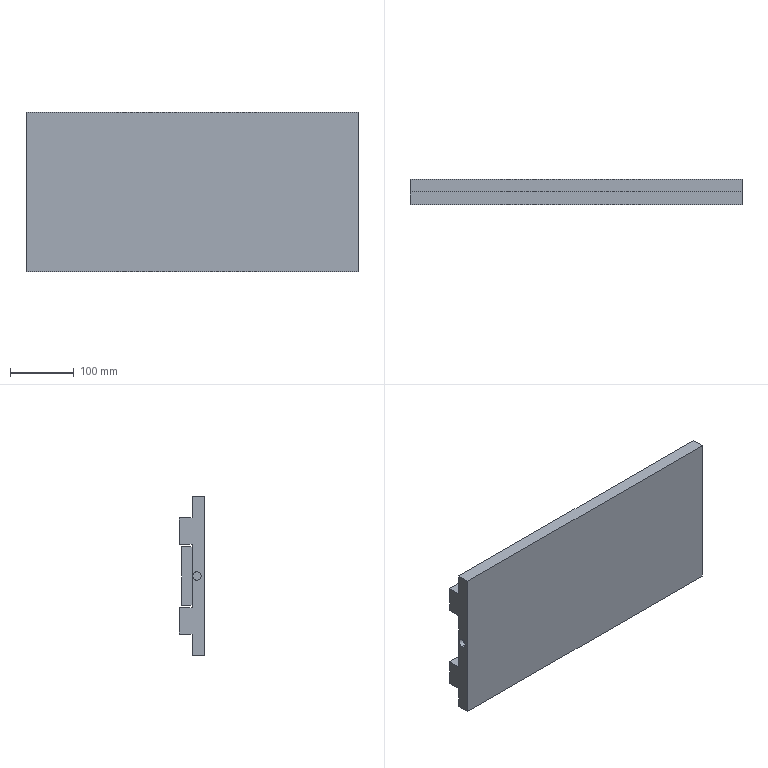Component | SolidWorks | X-AxisSupportBase-1 | 1 solid | 38 faces | box 520 x 40 x 250 mm | volume 3501982 mm3 | plane 26 | cylinder 12 | commonest cylinder face diameters 5.084 x8 13.093 x2 2.946 x2
STEP:
#1=COLOUR_RGB('',0.7922,0.8196,0.9333);
#2=FILL_AREA_STYLE_COLOUR('',#1);
#3=FILL_AREA_STYLE('',(#2));
#4=SURFACE_STYLE_FILL_AREA(#3);
#5=SURFACE_SIDE_STYLE('',(#4));
#6=SURFACE_STYLE_USAGE(.BOTH.,#5);
#7=PRESENTATION_STYLE_ASSIGNMENT((#6));
#8=CARTESIAN_POINT('',(6.767,1.417,1.368));
#9=VERTEX_POINT('',#8);
#10=CARTESIAN_POINT('',(6.767,1.417,1.568));
#11=VERTEX_POINT('',#10);
#12=CARTESIAN_POINT('',(6.767,1.417,1.468));
#13=DIRECTION('',(0.,1.,0.));
#14=DIRECTION('',(0.,0.,1.));
#15=AXIS2_PLACEMENT_3D('',#12,#13,#14);
#16=CIRCLE('',#15,0.1001);
#17=EDGE_CURVE('',#9,#11,#16,.T.);
#18=ORIENTED_EDGE('',*,*,#17,.T.);
#19=CARTESIAN_POINT('',(6.767,0.7874,1.568));
#20=VERTEX_POINT('',#19);
#21=CARTESIAN_POINT('',(6.767,1.417,1.568));
#22=DIRECTION('',(0.,-1.,0.));
#23=VECTOR('',#22,39.37);
#24=LINE('',#21,#23);
#25=EDGE_CURVE('',#11,#20,#24,.T.);
#26=ORIENTED_EDGE('',*,*,#25,.T.);
#27=CARTESIAN_POINT('',(6.767,0.7874,1.368));
#28=VERTEX_POINT('',#27);
#29=CARTESIAN_POINT('',(6.767,0.7874,1.468));
#30=DIRECTION('',(0.,1.,0.));
#31=DIRECTION('',(0.,0.,1.));
#32=AXIS2_PLACEMENT_3D('',#29,#30,#31);
#33=CIRCLE('',#32,0.1001);
#34=EDGE_CURVE('',#28,#20,#33,.T.);
#35=ORIENTED_EDGE('',*,*,#34,.F.);
#36=CARTESIAN_POINT('',(6.767,1.417,1.368));
#37=DIRECTION('',(0.,-1.,0.));
#38=VECTOR('',#37,39.37);
#39=LINE('',#36,#38);
#40=EDGE_CURVE('',#9,#28,#39,.T.);
#41=ORIENTED_EDGE('',*,*,#40,.F.);
#42=EDGE_LOOP('',(#18,#26,#35,#41));
#43=FACE_OUTER_BOUND('',#42,.T.);
#44=CARTESIAN_POINT('',(6.767,1.417,1.468));
#45=DIRECTION('',(0.,-1.,0.));
#46=DIRECTION('',(0.,0.,-1.));
#47=AXIS2_PLACEMENT_3D('',#44,#45,#46);
#48=CYLINDRICAL_SURFACE('',#47,0.1001);
#49=ADVANCED_FACE('',(#43),#48,.F.);
#50=CARTESIAN_POINT('',(6.208,1.417,1.368));
#51=VERTEX_POINT('',#50);
#52=CARTESIAN_POINT('',(6.208,1.417,1.568));
#53=VERTEX_POINT('',#52);
#54=CARTESIAN_POINT('',(6.208,1.417,1.468));
#55=DIRECTION('',(0.,1.,0.));
#56=DIRECTION('',(0.,0.,1.));
#57=AXIS2_PLACEMENT_3D('',#54,#55,#56);
#58=CIRCLE('',#57,0.1001);
#59=EDGE_CURVE('',#51,#53,#58,.T.);
#60=ORIENTED_EDGE('',*,*,#59,.T.);
#61=CARTESIAN_POINT('',(6.208,0.7874,1.568));
#62=VERTEX_POINT('',#61);
#63=CARTESIAN_POINT('',(6.208,1.417,1.568));
#64=DIRECTION('',(0.,-1.,0.));
#65=VECTOR('',#64,39.37);
#66=LINE('',#63,#65);
#67=EDGE_CURVE('',#53,#62,#66,.T.);
#68=ORIENTED_EDGE('',*,*,#67,.T.);
#69=CARTESIAN_POINT('',(6.208,0.7874,1.368));
#70=VERTEX_POINT('',#69);
#71=CARTESIAN_POINT('',(6.208,0.7874,1.468));
#72=DIRECTION('',(0.,1.,0.));
#73=DIRECTION('',(0.,0.,1.));
#74=AXIS2_PLACEMENT_3D('',#71,#72,#73);
#75=CIRCLE('',#74,0.1001);
#76=EDGE_CURVE('',#70,#62,#75,.T.);
#77=ORIENTED_EDGE('',*,*,#76,.F.);
#78=CARTESIAN_POINT('',(6.208,1.417,1.368));
#79=DIRECTION('',(0.,-1.,0.));
#80=VECTOR('',#79,39.37);
#81=LINE('',#78,#80);
#82=EDGE_CURVE('',#51,#70,#81,.T.);
#83=ORIENTED_EDGE('',*,*,#82,.F.);
#84=EDGE_LOOP('',(#60,#68,#77,#83));
#85=FACE_OUTER_BOUND('',#84,.T.);
#86=CARTESIAN_POINT('',(6.208,1.417,1.468));
#87=DIRECTION('',(0.,-1.,0.));
#88=DIRECTION('',(0.,0.,-1.));
#89=AXIS2_PLACEMENT_3D('',#86,#87,#88);
#90=CYLINDRICAL_SURFACE('',#89,0.1001);
#91=ADVANCED_FACE('',(#85),#90,.F.);
#92=CARTESIAN_POINT('',(6.767,1.417,-1.568));
#93=VERTEX_POINT('',#92);
#94=CARTESIAN_POINT('',(6.767,1.417,-1.368));
#95=VERTEX_POINT('',#94);
#96=CARTESIAN_POINT('',(6.767,1.417,-1.468));
#97=DIRECTION('',(0.,1.,0.));
#98=DIRECTION('',(0.,0.,1.));
#99=AXIS2_PLACEMENT_3D('',#96,#97,#98);
#100=CIRCLE('',#99,0.1001);
#101=EDGE_CURVE('',#93,#95,#100,.T.);
#102=ORIENTED_EDGE('',*,*,#101,.T.);
#103=CARTESIAN_POINT('',(6.767,0.7874,-1.368));
#104=VERTEX_POINT('',#103);
#105=CARTESIAN_POINT('',(6.767,1.417,-1.368));
#106=DIRECTION('',(0.,-1.,0.));
#107=VECTOR('',#106,39.37);
#108=LINE('',#105,#107);
#109=EDGE_CURVE('',#95,#104,#108,.T.);
#110=ORIENTED_EDGE('',*,*,#109,.T.);
#111=CARTESIAN_POINT('',(6.767,0.7874,-1.568));
#112=VERTEX_POINT('',#111);
#113=CARTESIAN_POINT('',(6.767,0.7874,-1.468));
#114=DIRECTION('',(0.,1.,0.));
#115=DIRECTION('',(0.,0.,1.));
#116=AXIS2_PLACEMENT_3D('',#113,#114,#115);
#117=CIRCLE('',#116,0.1001);
#118=EDGE_CURVE('',#112,#104,#117,.T.);
#119=ORIENTED_EDGE('',*,*,#118,.F.);
#120=CARTESIAN_POINT('',(6.767,1.417,-1.568));
#121=DIRECTION('',(0.,-1.,0.));
#122=VECTOR('',#121,39.37);
#123=LINE('',#120,#122);
#124=EDGE_CURVE('',#93,#112,#123,.T.);
#125=ORIENTED_EDGE('',*,*,#124,.F.);
#126=EDGE_LOOP('',(#102,#110,#119,#125));
#127=FACE_OUTER_BOUND('',#126,.T.);
#128=CARTESIAN_POINT('',(6.767,1.417,-1.468));
#129=DIRECTION('',(0.,-1.,0.));
#130=DIRECTION('',(0.,0.,-1.));
#131=AXIS2_PLACEMENT_3D('',#128,#129,#130);
#132=CYLINDRICAL_SURFACE('',#131,0.1001);
#133=ADVANCED_FACE('',(#127),#132,.F.);
#134=CARTESIAN_POINT('',(6.208,1.417,-1.568));
#135=VERTEX_POINT('',#134);
#136=CARTESIAN_POINT('',(6.208,1.417,-1.368));
#137=VERTEX_POINT('',#136);
#138=CARTESIAN_POINT('',(6.208,1.417,-1.468));
#139=DIRECTION('',(0.,1.,0.));
#140=DIRECTION('',(0.,0.,1.));
#141=AXIS2_PLACEMENT_3D('',#138,#139,#140);
#142=CIRCLE('',#141,0.1001);
#143=EDGE_CURVE('',#135,#137,#142,.T.);
#144=ORIENTED_EDGE('',*,*,#143,.T.);
#145=CARTESIAN_POINT('',(6.208,0.7874,-1.368));
#146=VERTEX_POINT('',#145);
#147=CARTESIAN_POINT('',(6.208,1.417,-1.368));
#148=DIRECTION('',(0.,-1.,0.));
#149=VECTOR('',#148,39.37);
#150=LINE('',#147,#149);
#151=EDGE_CURVE('',#137,#146,#150,.T.);
#152=ORIENTED_EDGE('',*,*,#151,.T.);
#153=CARTESIAN_POINT('',(6.208,0.7874,-1.568));
#154=VERTEX_POINT('',#153);
#155=CARTESIAN_POINT('',(6.208,0.7874,-1.468));
#156=DIRECTION('',(0.,1.,0.));
#157=DIRECTION('',(0.,0.,1.));
#158=AXIS2_PLACEMENT_3D('',#155,#156,#157);
#159=CIRCLE('',#158,0.1001);
#160=EDGE_CURVE('',#154,#146,#159,.T.);
#161=ORIENTED_EDGE('',*,*,#160,.F.);
#162=CARTESIAN_POINT('',(6.208,1.417,-1.568));
#163=DIRECTION('',(0.,-1.,0.));
#164=VECTOR('',#163,39.37);
#165=LINE('',#162,#164);
#166=EDGE_CURVE('',#135,#154,#165,.T.);
#167=ORIENTED_EDGE('',*,*,#166,.F.);
#168=EDGE_LOOP('',(#144,#152,#161,#167));
#169=FACE_OUTER_BOUND('',#168,.T.);
#170=CARTESIAN_POINT('',(6.208,1.417,-1.468));
#171=DIRECTION('',(0.,-1.,0.));
#172=DIRECTION('',(0.,0.,-1.));
#173=AXIS2_PLACEMENT_3D('',#170,#171,#172);
#174=CYLINDRICAL_SURFACE('',#173,0.1001);
#175=ADVANCED_FACE('',(#169),#174,.F.);
#176=CARTESIAN_POINT('',(-10.591,0.4812,-0.2577));
#177=VERTEX_POINT('',#176);
#178=CARTESIAN_POINT('',(-10.591,0.4812,0.2577));
#179=VERTEX_POINT('',#178);
#180=CARTESIAN_POINT('',(-10.591,0.4812,0.));
#181=DIRECTION('',(-1.,0.,0.));
#182=DIRECTION('',(0.,0.,1.));
#183=AXIS2_PLACEMENT_3D('',#180,#181,#182);
#184=CIRCLE('',#183,0.2577);
#185=EDGE_CURVE('',#177,#179,#184,.T.);
#186=ORIENTED_EDGE('',*,*,#185,.F.);
#187=CARTESIAN_POINT('',(-10.906,0.4812,-0.2577));
#188=VERTEX_POINT('',#187);
#189=CARTESIAN_POINT('',(-10.591,0.4812,-0.2577));
#190=DIRECTION('',(-1.,0.,0.));
#191=VECTOR('',#190,39.37);
#192=LINE('',#189,#191);
#193=EDGE_CURVE('',#177,#188,#192,.T.);
#194=ORIENTED_EDGE('',*,*,#193,.T.);
#195=CARTESIAN_POINT('',(-10.906,0.4812,0.2577));
#196=VERTEX_POINT('',#195);
#197=CARTESIAN_POINT('',(-10.906,0.4812,0.));
#198=DIRECTION('',(-1.,0.,0.));
#199=DIRECTION('',(0.,0.,1.));
#200=AXIS2_PLACEMENT_3D('',#197,#198,#199);
#201=CIRCLE('',#200,0.2577);
#202=EDGE_CURVE('',#188,#196,#201,.T.);
#203=ORIENTED_EDGE('',*,*,#202,.T.);
#204=CARTESIAN_POINT('',(-10.591,0.4812,0.2577));
#205=DIRECTION('',(-1.,0.,0.));
#206=VECTOR('',#205,39.37);
#207=LINE('',#204,#206);
#208=EDGE_CURVE('',#179,#196,#207,.T.);
#209=ORIENTED_EDGE('',*,*,#208,.F.);
#210=EDGE_LOOP('',(#186,#194,#203,#209));
#211=FACE_OUTER_BOUND('',#210,.T.);
#212=CARTESIAN_POINT('',(-10.591,0.4812,0.));
#213=DIRECTION('',(-1.,0.,0.));
#214=DIRECTION('',(0.,0.,1.));
#215=AXIS2_PLACEMENT_3D('',#212,#213,#214);
#216=CYLINDRICAL_SURFACE('',#215,0.2577);
#217=ADVANCED_FACE('',(#211),#216,.F.);
#218=CARTESIAN_POINT('',(-10.906,1.575,3.579));
#219=VERTEX_POINT('',#218);
#220=CARTESIAN_POINT('',(9.567,1.575,3.579));
#221=VERTEX_POINT('',#220);
#222=CARTESIAN_POINT('',(0.,1.575,3.579));
#223=DIRECTION('',(1.,0.,0.));
#224=VECTOR('',#223,39.37);
#225=LINE('',#222,#224);
#226=EDGE_CURVE('',#219,#221,#225,.T.);
#227=ORIENTED_EDGE('',*,*,#226,.T.);
#228=CARTESIAN_POINT('',(9.567,1.575,1.945));
#229=VERTEX_POINT('',#228);
#230=CARTESIAN_POINT('',(9.567,1.575,0.));
#231=DIRECTION('',(0.,0.,-1.));
#232=VECTOR('',#231,39.37);
#233=LINE('',#230,#232);
#234=EDGE_CURVE('',#221,#229,#233,.T.);
#235=ORIENTED_EDGE('',*,*,#234,.T.);
#236=CARTESIAN_POINT('',(-10.906,1.575,1.945));
#237=VERTEX_POINT('',#236);
#238=CARTESIAN_POINT('',(0.,1.575,1.945));
#239=DIRECTION('',(-1.,0.,0.));
#240=VECTOR('',#239,39.37);
#241=LINE('',#238,#240);
#242=EDGE_CURVE('',#229,#237,#241,.T.);
#243=ORIENTED_EDGE('',*,*,#242,.T.);
#244=CARTESIAN_POINT('',(-10.906,1.575,0.));
#245=DIRECTION('',(0.,0.,1.));
#246=VECTOR('',#245,39.37);
#247=LINE('',#244,#246);
#248=EDGE_CURVE('',#237,#219,#247,.T.);
#249=ORIENTED_EDGE('',*,*,#248,.T.);
#250=EDGE_LOOP('',(#227,#235,#243,#249));
#251=FACE_OUTER_BOUND('',#250,.T.);
#252=CARTESIAN_POINT('',(0.,1.575,0.));
#253=DIRECTION('',(0.,1.,0.));
#254=DIRECTION('',(0.,0.,1.));
#255=AXIS2_PLACEMENT_3D('',#252,#253,#254);
#256=PLANE('',#255);
#257=ADVANCED_FACE('',(#251),#256,.T.);
#258=CARTESIAN_POINT('',(9.567,0.7874,3.579));
#259=VERTEX_POINT('',#258);
#260=CARTESIAN_POINT('',(9.567,0.7874,4.921));
#261=VERTEX_POINT('',#260);
#262=CARTESIAN_POINT('',(9.567,0.7874,0.));
#263=DIRECTION('',(0.,0.,1.));
#264=VECTOR('',#263,39.37);
#265=LINE('',#262,#264);
#266=EDGE_CURVE('',#259,#261,#265,.T.);
#267=ORIENTED_EDGE('',*,*,#266,.F.);
#268=CARTESIAN_POINT('',(-10.906,0.7874,3.579));
#269=VERTEX_POINT('',#268);
#270=CARTESIAN_POINT('',(0.,0.7874,3.579));
#271=DIRECTION('',(1.,0.,0.));
#272=VECTOR('',#271,39.37);
#273=LINE('',#270,#272);
#274=EDGE_CURVE('',#269,#259,#273,.T.);
#275=ORIENTED_EDGE('',*,*,#274,.F.);
#276=CARTESIAN_POINT('',(-10.906,0.7874,4.921));
#277=VERTEX_POINT('',#276);
#278=CARTESIAN_POINT('',(-10.906,0.7874,4.528));
#279=DIRECTION('',(0.,0.,1.));
#280=VECTOR('',#279,39.37);
#281=LINE('',#278,#280);
#282=EDGE_CURVE('',#269,#277,#281,.T.);
#283=ORIENTED_EDGE('',*,*,#282,.T.);
#284=CARTESIAN_POINT('',(10.906,0.7874,4.921));
#285=DIRECTION('',(-1.,0.,0.));
#286=VECTOR('',#285,39.37);
#287=LINE('',#284,#286);
#288=EDGE_CURVE('',#261,#277,#287,.T.);
#289=ORIENTED_EDGE('',*,*,#288,.F.);
#290=EDGE_LOOP('',(#267,#275,#283,#289));
#291=FACE_OUTER_BOUND('',#290,.T.);
#292=CARTESIAN_POINT('',(0.,0.7874,0.));
#293=DIRECTION('',(0.,-1.,0.));
#294=DIRECTION('',(0.,0.,-1.));
#295=AXIS2_PLACEMENT_3D('',#292,#293,#294);
#296=PLANE('',#295);
#297=ADVANCED_FACE('',(#291),#296,.F.);
#298=CARTESIAN_POINT('',(9.567,0.7874,-4.921));
#299=VERTEX_POINT('',#298);
#300=CARTESIAN_POINT('',(9.567,0.7874,-3.579));
#301=VERTEX_POINT('',#300);
#302=CARTESIAN_POINT('',(9.567,0.7874,0.));
#303=DIRECTION('',(0.,0.,1.));
#304=VECTOR('',#303,39.37);
#305=LINE('',#302,#304);
#306=EDGE_CURVE('',#299,#301,#305,.T.);
#307=ORIENTED_EDGE('',*,*,#306,.F.);
#308=CARTESIAN_POINT('',(-10.906,0.7874,-4.921));
#309=VERTEX_POINT('',#308);
#310=CARTESIAN_POINT('',(-10.906,0.7874,-4.921));
#311=DIRECTION('',(1.,0.,0.));
#312=VECTOR('',#311,39.37);
#313=LINE('',#310,#312);
#314=EDGE_CURVE('',#309,#299,#313,.T.);
#315=ORIENTED_EDGE('',*,*,#314,.F.);
#316=CARTESIAN_POINT('',(-10.906,0.7874,-3.579));
#317=VERTEX_POINT('',#316);
#318=CARTESIAN_POINT('',(-10.906,0.7874,4.528));
#319=DIRECTION('',(0.,0.,1.));
#320=VECTOR('',#319,39.37);
#321=LINE('',#318,#320);
#322=EDGE_CURVE('',#309,#317,#321,.T.);
#323=ORIENTED_EDGE('',*,*,#322,.T.);
#324=CARTESIAN_POINT('',(0.,0.7874,-3.579));
#325=DIRECTION('',(1.,0.,0.));
#326=VECTOR('',#325,39.37);
#327=LINE('',#324,#326);
#328=EDGE_CURVE('',#317,#301,#327,.T.);
#329=ORIENTED_EDGE('',*,*,#328,.T.);
#330=EDGE_LOOP('',(#307,#315,#323,#329));
#331=FACE_OUTER_BOUND('',#330,.T.);
#332=CARTESIAN_POINT('',(0.,0.7874,0.));
#333=DIRECTION('',(0.,-1.,0.));
#334=DIRECTION('',(0.,0.,-1.));
#335=AXIS2_PLACEMENT_3D('',#332,#333,#334);
#336=PLANE('',#335);
#337=ADVANCED_FACE('',(#331),#336,.F.);
#338=CARTESIAN_POINT('',(9.567,0.,-4.921));
#339=VERTEX_POINT('',#338);
#340=CARTESIAN_POINT('',(-10.906,0.,-4.921));
#341=VERTEX_POINT('',#340);
#342=CARTESIAN_POINT('',(10.906,0.,-4.921));
#343=DIRECTION('',(-1.,0.,0.));
#344=VECTOR('',#343,39.37);
#345=LINE('',#342,#344);
#346=EDGE_CURVE('',#339,#341,#345,.T.);
#347=ORIENTED_EDGE('',*,*,#346,.F.);
#348=CARTESIAN_POINT('',(9.567,0.,4.921));
#349=VERTEX_POINT('',#348);
#350=CARTESIAN_POINT('',(9.567,0.,0.));
#351=DIRECTION('',(0.,0.,-1.));
#352=VECTOR('',#351,39.37);
#353=LINE('',#350,#352);
#354=EDGE_CURVE('',#349,#339,#353,.T.);
#355=ORIENTED_EDGE('',*,*,#354,.F.);
#356=CARTESIAN_POINT('',(-10.906,0.,4.921));
#357=VERTEX_POINT('',#356);
#358=CARTESIAN_POINT('',(-10.906,0.,4.921));
#359=DIRECTION('',(1.,0.,0.));
#360=VECTOR('',#359,39.37);
#361=LINE('',#358,#360);
#362=EDGE_CURVE('',#357,#349,#361,.T.);
#363=ORIENTED_EDGE('',*,*,#362,.F.);
#364=CARTESIAN_POINT('',(-10.906,0.,4.528));
#365=DIRECTION('',(0.,0.,1.));
#366=VECTOR('',#365,39.37);
#367=LINE('',#364,#366);
#368=EDGE_CURVE('',#341,#357,#367,.T.);
#369=ORIENTED_EDGE('',*,*,#368,.F.);
#370=EDGE_LOOP('',(#347,#355,#363,#369));
#371=FACE_OUTER_BOUND('',#370,.T.);
#372=CARTESIAN_POINT('',(0.,0.,0.));
#373=DIRECTION('',(0.,-1.,0.));
#374=DIRECTION('',(0.,0.,-1.));
#375=AXIS2_PLACEMENT_3D('',#372,#373,#374);
#376=PLANE('',#375);
#377=ADVANCED_FACE('',(#371),#376,.T.);
#378=CARTESIAN_POINT('',(-10.906,1.575,-3.579));
#379=VERTEX_POINT('',#378);
#380=CARTESIAN_POINT('',(9.567,1.575,-3.579));
#381=VERTEX_POINT('',#380);
#382=CARTESIAN_POINT('',(0.,1.575,-3.579));
#383=DIRECTION('',(1.,0.,0.));
#384=VECTOR('',#383,39.37);
#385=LINE('',#382,#384);
#386=EDGE_CURVE('',#379,#381,#385,.T.);
#387=ORIENTED_EDGE('',*,*,#386,.T.);
#388=CARTESIAN_POINT('',(9.567,1.575,-3.579));
#389=DIRECTION('',(0.,-1.,0.));
#390=VECTOR('',#389,39.37);
#391=LINE('',#388,#390);
#392=EDGE_CURVE('',#381,#301,#391,.T.);
#393=ORIENTED_EDGE('',*,*,#392,.T.);
#394=ORIENTED_EDGE('',*,*,#328,.F.);
#395=CARTESIAN_POINT('',(-10.906,1.575,-3.579));
#396=DIRECTION('',(0.,-1.,0.));
#397=VECTOR('',#396,39.37);
#398=LINE('',#395,#397);
#399=EDGE_CURVE('',#379,#317,#398,.T.);
#400=ORIENTED_EDGE('',*,*,#399,.F.);
#401=EDGE_LOOP('',(#387,#393,#394,#400));
#402=FACE_OUTER_BOUND('',#401,.T.);
#403=CARTESIAN_POINT('',(0.,1.575,-3.579));
#404=DIRECTION('',(0.,0.,-1.));
#405=DIRECTION('',(-1.,0.,0.));
#406=AXIS2_PLACEMENT_3D('',#403,#404,#405);
#407=PLANE('',#406);
#408=ADVANCED_FACE('',(#402),#407,.T.);
#409=CARTESIAN_POINT('',(9.567,1.575,-1.945));
#410=VERTEX_POINT('',#409);
#411=CARTESIAN_POINT('',(-10.906,1.575,-1.945));
#412=VERTEX_POINT('',#411);
#413=CARTESIAN_POINT('',(0.,1.575,-1.945));
#414=DIRECTION('',(-1.,0.,0.));
#415=VECTOR('',#414,39.37);
#416=LINE('',#413,#415);
#417=EDGE_CURVE('',#410,#412,#416,.T.);
#418=ORIENTED_EDGE('',*,*,#417,.F.);
#419=CARTESIAN_POINT('',(9.567,1.575,0.));
#420=DIRECTION('',(0.,0.,-1.));
#421=VECTOR('',#420,39.37);
#422=LINE('',#419,#421);
#423=EDGE_CURVE('',#410,#381,#422,.T.);
#424=ORIENTED_EDGE('',*,*,#423,.T.);
#425=ORIENTED_EDGE('',*,*,#386,.F.);
#426=CARTESIAN_POINT('',(-10.906,1.575,0.));
#427=DIRECTION('',(0.,0.,1.));
#428=VECTOR('',#427,39.37);
#429=LINE('',#426,#428);
#430=EDGE_CURVE('',#379,#412,#429,.T.);
#431=ORIENTED_EDGE('',*,*,#430,.T.);
#432=EDGE_LOOP('',(#418,#424,#425,#431));
#433=FACE_OUTER_BOUND('',#432,.T.);
#434=CARTESIAN_POINT('',(0.,1.575,0.));
#435=DIRECTION('',(0.,1.,0.));
#436=DIRECTION('',(0.,0.,1.));
#437=AXIS2_PLACEMENT_3D('',#434,#435,#436);
#438=PLANE('',#437);
#439=ADVANCED_FACE('',(#433),#438,.T.);
#440=CARTESIAN_POINT('',(9.567,1.575,3.579));
#441=DIRECTION('',(0.,-1.,0.));
#442=VECTOR('',#441,39.37);
#443=LINE('',#440,#442);
#444=EDGE_CURVE('',#221,#259,#443,.T.);
#445=ORIENTED_EDGE('',*,*,#444,.F.);
#446=ORIENTED_EDGE('',*,*,#226,.F.);
#447=CARTESIAN_POINT('',(-10.906,1.575,3.579));
#448=DIRECTION('',(0.,-1.,0.));
#449=VECTOR('',#448,39.37);
#450=LINE('',#447,#449);
#451=EDGE_CURVE('',#219,#269,#450,.T.);
#452=ORIENTED_EDGE('',*,*,#451,.T.);
#453=ORIENTED_EDGE('',*,*,#274,.T.);
#454=EDGE_LOOP('',(#445,#446,#452,#453));
#455=FACE_OUTER_BOUND('',#454,.T.);
#456=CARTESIAN_POINT('',(0.,1.575,3.579));
#457=DIRECTION('',(0.,0.,-1.));
#458=DIRECTION('',(-1.,0.,0.));
#459=AXIS2_PLACEMENT_3D('',#456,#457,#458);
#460=PLANE('',#459);
#461=ADVANCED_FACE('',(#455),#460,.F.);
#462=CARTESIAN_POINT('',(9.567,0.8454,-1.945));
#463=VERTEX_POINT('',#462);
#464=CARTESIAN_POINT('',(9.567,0.7952,-1.916));
#465=VERTEX_POINT('',#464);
#466=CARTESIAN_POINT('',(9.567,0.8454,-1.887));
#467=DIRECTION('',(-1.,0.,0.));
#468=DIRECTION('',(0.,0.,-1.));
#469=AXIS2_PLACEMENT_3D('',#466,#467,#468);
#470=CIRCLE('',#469,0.058);
#471=EDGE_CURVE('',#463,#465,#470,.T.);
#472=ORIENTED_EDGE('',*,*,#471,.F.);
#473=CARTESIAN_POINT('',(-10.906,0.8454,-1.945));
#474=VERTEX_POINT('',#473);
#475=CARTESIAN_POINT('',(19.803,0.8454,-1.945));
#476=DIRECTION('',(-1.,0.,0.));
#477=VECTOR('',#476,39.37);
#478=LINE('',#475,#477);
#479=EDGE_CURVE('',#463,#474,#478,.T.);
#480=ORIENTED_EDGE('',*,*,#479,.T.);
#481=CARTESIAN_POINT('',(-10.906,0.7952,-1.916));
#482=VERTEX_POINT('',#481);
#483=CARTESIAN_POINT('',(-10.906,0.8454,-1.887));
#484=DIRECTION('',(-1.,0.,0.));
#485=DIRECTION('',(0.,0.,1.));
#486=AXIS2_PLACEMENT_3D('',#483,#484,#485);
#487=CIRCLE('',#486,0.058);
#488=EDGE_CURVE('',#474,#482,#487,.T.);
#489=ORIENTED_EDGE('',*,*,#488,.T.);
#490=CARTESIAN_POINT('',(19.803,0.7952,-1.916));
#491=DIRECTION('',(-1.,0.,0.));
#492=VECTOR('',#491,39.37);
#493=LINE('',#490,#492);
#494=EDGE_CURVE('',#465,#482,#493,.T.);
#495=ORIENTED_EDGE('',*,*,#494,.F.);
#496=EDGE_LOOP('',(#472,#480,#489,#495));
#497=FACE_OUTER_BOUND('',#496,.T.);
#498=CARTESIAN_POINT('',(19.803,0.8454,-1.887));
#499=DIRECTION('',(-1.,0.,0.));
#500=DIRECTION('',(0.,0.,1.));
#501=AXIS2_PLACEMENT_3D('',#498,#499,#500);
#502=CYLINDRICAL_SURFACE('',#501,0.058);
#503=ADVANCED_FACE('',(#497),#502,.F.);
#504=CARTESIAN_POINT('',(9.567,0.,-1.945));
#505=DIRECTION('',(0.,-1.,-0.));
#506=VECTOR('',#505,39.37);
#507=LINE('',#504,#506);
#508=EDGE_CURVE('',#410,#463,#507,.T.);
#509=ORIENTED_EDGE('',*,*,#508,.F.);
#510=ORIENTED_EDGE('',*,*,#417,.T.);
#511=CARTESIAN_POINT('',(-10.906,0.,-1.945));
#512=DIRECTION('',(0.,-1.,-0.));
#513=VECTOR('',#512,39.37);
#514=LINE('',#511,#513);
#515=EDGE_CURVE('',#412,#474,#514,.T.);
#516=ORIENTED_EDGE('',*,*,#515,.T.);
#517=ORIENTED_EDGE('',*,*,#479,.F.);
#518=EDGE_LOOP('',(#509,#510,#516,#517));
#519=FACE_OUTER_BOUND('',#518,.T.);
#520=CARTESIAN_POINT('',(19.803,0.,-1.945));
#521=DIRECTION('',(0.,0.,-1.));
#522=DIRECTION('',(0.,1.,0.));
#523=AXIS2_PLACEMENT_3D('',#520,#521,#522);
#524=PLANE('',#523);
#525=ADVANCED_FACE('',(#519),#524,.F.);
#526=CARTESIAN_POINT('',(9.567,0.8454,1.945));
#527=VERTEX_POINT('',#526);
#528=CARTESIAN_POINT('',(-10.906,0.8454,1.945));
#529=VERTEX_POINT('',#528);
#530=CARTESIAN_POINT('',(19.803,0.8454,1.945));
#531=DIRECTION('',(-1.,0.,0.));
#532=VECTOR('',#531,39.37);
#533=LINE('',#530,#532);
#534=EDGE_CURVE('',#527,#529,#533,.T.);
#535=ORIENTED_EDGE('',*,*,#534,.F.);
#536=CARTESIAN_POINT('',(9.567,0.7952,1.916));
#537=VERTEX_POINT('',#536);
#538=CARTESIAN_POINT('',(9.567,0.8454,1.887));
#539=DIRECTION('',(1.,0.,0.));
#540=DIRECTION('',(0.,0.,-1.));
#541=AXIS2_PLACEMENT_3D('',#538,#539,#540);
#542=CIRCLE('',#541,0.058);
#543=EDGE_CURVE('',#527,#537,#542,.T.);
#544=ORIENTED_EDGE('',*,*,#543,.T.);
#545=CARTESIAN_POINT('',(-10.906,0.7952,1.916));
#546=VERTEX_POINT('',#545);
#547=CARTESIAN_POINT('',(19.803,0.7952,1.916));
#548=DIRECTION('',(-1.,0.,0.));
#549=VECTOR('',#548,39.37);
#550=LINE('',#547,#549);
#551=EDGE_CURVE('',#537,#546,#550,.T.);
#552=ORIENTED_EDGE('',*,*,#551,.T.);
#553=CARTESIAN_POINT('',(-10.906,0.8454,1.887));
#554=DIRECTION('',(1.,0.,0.));
#555=DIRECTION('',(0.,0.,-1.));
#556=AXIS2_PLACEMENT_3D('',#553,#554,#555);
#557=CIRCLE('',#556,0.058);
#558=EDGE_CURVE('',#529,#546,#557,.T.);
#559=ORIENTED_EDGE('',*,*,#558,.F.);
#560=EDGE_LOOP('',(#535,#544,#552,#559));
#561=FACE_OUTER_BOUND('',#560,.T.);
#562=CARTESIAN_POINT('',(19.803,0.8454,1.887));
#563=DIRECTION('',(-1.,0.,0.));
#564=DIRECTION('',(0.,0.,1.));
#565=AXIS2_PLACEMENT_3D('',#562,#563,#564);
#566=CYLINDRICAL_SURFACE('',#565,0.058);
#567=ADVANCED_FACE('',(#561),#566,.F.);
#568=ORIENTED_EDGE('',*,*,#242,.F.);
#569=CARTESIAN_POINT('',(9.567,0.,1.945));
#570=DIRECTION('',(0.,-1.,0.));
#571=VECTOR('',#570,39.37);
#572=LINE('',#569,#571);
#573=EDGE_CURVE('',#229,#527,#572,.T.);
#574=ORIENTED_EDGE('',*,*,#573,.T.);
#575=ORIENTED_EDGE('',*,*,#534,.T.);
#576=CARTESIAN_POINT('',(-10.906,0.,1.945));
#577=DIRECTION('',(0.,-1.,0.));
#578=VECTOR('',#577,39.37);
#579=LINE('',#576,#578);
#580=EDGE_CURVE('',#237,#529,#579,.T.);
#581=ORIENTED_EDGE('',*,*,#580,.F.);
#582=EDGE_LOOP('',(#568,#574,#575,#581));
#583=FACE_OUTER_BOUND('',#582,.T.);
#584=CARTESIAN_POINT('',(19.803,0.,1.945));
#585=DIRECTION('',(0.,-0.,-1.));
#586=DIRECTION('',(0.,1.,-0.));
#587=AXIS2_PLACEMENT_3D('',#584,#585,#586);
#588=PLANE('',#587);
#589=ADVANCED_FACE('',(#583),#588,.T.);
#590=ORIENTED_EDGE('',*,*,#362,.T.);
#591=CARTESIAN_POINT('',(9.567,0.,4.921));
#592=DIRECTION('',(0.,1.,0.));
#593=VECTOR('',#592,39.37);
#594=LINE('',#591,#593);
#595=EDGE_CURVE('',#349,#261,#594,.T.);
#596=ORIENTED_EDGE('',*,*,#595,.T.);
#597=ORIENTED_EDGE('',*,*,#288,.T.);
#598=CARTESIAN_POINT('',(-10.906,0.7874,4.921));
#599=DIRECTION('',(0.,-1.,0.));
#600=VECTOR('',#599,39.37);
#601=LINE('',#598,#600);
#602=EDGE_CURVE('',#277,#357,#601,.T.);
#603=ORIENTED_EDGE('',*,*,#602,.T.);
#604=EDGE_LOOP('',(#590,#596,#597,#603));
#605=FACE_OUTER_BOUND('',#604,.T.);
#606=CARTESIAN_POINT('',(0.,0.,4.921));
#607=DIRECTION('',(0.,0.,1.));
#608=DIRECTION('',(1.,0.,0.));
#609=AXIS2_PLACEMENT_3D('',#606,#607,#608);
#610=PLANE('',#609);
#611=ADVANCED_FACE('',(#605),#610,.T.);
#612=ORIENTED_EDGE('',*,*,#314,.T.);
#613=CARTESIAN_POINT('',(9.567,0.,-4.921));
#614=DIRECTION('',(0.,1.,0.));
#615=VECTOR('',#614,39.37);
#616=LINE('',#613,#615);
#617=EDGE_CURVE('',#339,#299,#616,.T.);
#618=ORIENTED_EDGE('',*,*,#617,.F.);
#619=ORIENTED_EDGE('',*,*,#346,.T.);
#620=CARTESIAN_POINT('',(-10.906,0.,-4.921));
#621=DIRECTION('',(0.,1.,0.));
#622=VECTOR('',#621,39.37);
#623=LINE('',#620,#622);
#624=EDGE_CURVE('',#341,#309,#623,.T.);
#625=ORIENTED_EDGE('',*,*,#624,.T.);
#626=EDGE_LOOP('',(#612,#618,#619,#625));
#627=FACE_OUTER_BOUND('',#626,.T.);
#628=CARTESIAN_POINT('',(0.,0.,-4.921));
#629=DIRECTION('',(0.,0.,-1.));
#630=DIRECTION('',(-1.,0.,0.));
#631=AXIS2_PLACEMENT_3D('',#628,#629,#630);
#632=PLANE('',#631);
#633=ADVANCED_FACE('',(#627),#632,.T.);
#634=CARTESIAN_POINT('',(7.039,0.7874,-1.791));
#635=VERTEX_POINT('',#634);
#636=CARTESIAN_POINT('',(5.936,0.7874,-1.791));
#637=VERTEX_POINT('',#636);
#638=CARTESIAN_POINT('',(7.039,0.7874,-1.791));
#639=DIRECTION('',(-1.,0.,-0.));
#640=VECTOR('',#639,39.37);
#641=LINE('',#638,#640);
#642=EDGE_CURVE('',#635,#637,#641,.T.);
#643=ORIENTED_EDGE('',*,*,#642,.F.);
#644=CARTESIAN_POINT('',(7.039,0.7874,1.791));
#645=VERTEX_POINT('',#644);
#646=CARTESIAN_POINT('',(7.039,0.7874,1.791));
#647=DIRECTION('',(0.,0.,-1.));
#648=VECTOR('',#647,39.37);
#649=LINE('',#646,#648);
#650=EDGE_CURVE('',#645,#635,#649,.T.);
#651=ORIENTED_EDGE('',*,*,#650,.F.);
#652=CARTESIAN_POINT('',(5.936,0.7874,1.791));
#653=VERTEX_POINT('',#652);
#654=CARTESIAN_POINT('',(5.936,0.7874,1.791));
#655=DIRECTION('',(1.,0.,0.));
#656=VECTOR('',#655,39.37);
#657=LINE('',#654,#656);
#658=EDGE_CURVE('',#653,#645,#657,.T.);
#659=ORIENTED_EDGE('',*,*,#658,.F.);
#660=CARTESIAN_POINT('',(5.936,0.7874,1.083));
#661=DIRECTION('',(0.,0.,1.));
#662=VECTOR('',#661,39.37);
#663=LINE('',#660,#662);
#664=EDGE_CURVE('',#637,#653,#663,.T.);
#665=ORIENTED_EDGE('',*,*,#664,.F.);
#666=EDGE_LOOP('',(#643,#651,#659,#665));
#667=FACE_BOUND('',#666,.T.);
#668=CARTESIAN_POINT('',(-10.906,0.7874,1.916));
#669=VERTEX_POINT('',#668);
#670=CARTESIAN_POINT('',(9.567,0.7874,1.916));
#671=VERTEX_POINT('',#670);
#672=CARTESIAN_POINT('',(0.,0.7874,1.916));
#673=DIRECTION('',(1.,0.,0.));
#674=VECTOR('',#673,39.37);
#675=LINE('',#672,#674);
#676=EDGE_CURVE('',#669,#671,#675,.T.);
#677=ORIENTED_EDGE('',*,*,#676,.T.);
#678=CARTESIAN_POINT('',(9.567,0.7874,-1.916));
#679=VERTEX_POINT('',#678);
#680=CARTESIAN_POINT('',(9.567,0.7874,1.916));
#681=DIRECTION('',(-0.,0.,-1.));
#682=VECTOR('',#681,39.37);
#683=LINE('',#680,#682);
#684=EDGE_CURVE('',#671,#679,#683,.T.);
#685=ORIENTED_EDGE('',*,*,#684,.T.);
#686=CARTESIAN_POINT('',(-10.906,0.7874,-1.916));
#687=VERTEX_POINT('',#686);
#688=CARTESIAN_POINT('',(0.,0.7874,-1.916));
#689=DIRECTION('',(1.,0.,0.));
#690=VECTOR('',#689,39.37);
#691=LINE('',#688,#690);
#692=EDGE_CURVE('',#687,#679,#691,.T.);
#693=ORIENTED_EDGE('',*,*,#692,.F.);
#694=CARTESIAN_POINT('',(-10.906,0.7874,4.528));
#695=DIRECTION('',(0.,0.,1.));
#696=VECTOR('',#695,39.37);
#697=LINE('',#694,#696);
#698=EDGE_CURVE('',#687,#669,#697,.T.);
#699=ORIENTED_EDGE('',*,*,#698,.T.);
#700=EDGE_LOOP('',(#677,#685,#693,#699));
#701=FACE_OUTER_BOUND('',#700,.T.);
#702=CARTESIAN_POINT('',(0.,0.7874,0.));
#703=DIRECTION('',(0.,-1.,0.));
#704=DIRECTION('',(0.,0.,-1.));
#705=AXIS2_PLACEMENT_3D('',#702,#703,#704);
#706=PLANE('',#705);
#707=ADVANCED_FACE('',(#667,#701),#706,.F.);
#708=ORIENTED_EDGE('',*,*,#692,.T.);
#709=CARTESIAN_POINT('',(9.567,-3.383,-1.916));
#710=DIRECTION('',(0.,1.,0.));
#711=VECTOR('',#710,39.37);
#712=LINE('',#709,#711);
#713=EDGE_CURVE('',#679,#465,#712,.T.);
#714=ORIENTED_EDGE('',*,*,#713,.T.);
#715=ORIENTED_EDGE('',*,*,#494,.T.);
#716=CARTESIAN_POINT('',(-10.906,1.575,-1.916));
#717=DIRECTION('',(0.,-1.,0.));
#718=VECTOR('',#717,39.37);
#719=LINE('',#716,#718);
#720=EDGE_CURVE('',#482,#687,#719,.T.);
#721=ORIENTED_EDGE('',*,*,#720,.T.);
#722=EDGE_LOOP('',(#708,#714,#715,#721));
#723=FACE_OUTER_BOUND('',#722,.T.);
#724=CARTESIAN_POINT('',(0.,1.575,-1.916));
#725=DIRECTION('',(0.,0.,-1.));
#726=DIRECTION('',(-1.,0.,0.));
#727=AXIS2_PLACEMENT_3D('',#724,#725,#726);
#728=PLANE('',#727);
#729=ADVANCED_FACE('',(#723),#728,.F.);
#730=CARTESIAN_POINT('',(-10.906,0.4812,0.));
#731=DIRECTION('',(-1.,0.,0.));
#732=DIRECTION('',(0.,0.,1.));
#733=AXIS2_PLACEMENT_3D('',#730,#731,#732);
#734=CIRCLE('',#733,0.2577);
#735=EDGE_CURVE('',#196,#188,#734,.T.);
#736=ORIENTED_EDGE('',*,*,#735,.F.);
#737=ORIENTED_EDGE('',*,*,#202,.F.);
#738=EDGE_LOOP('',(#736,#737));
#739=FACE_BOUND('',#738,.T.);
#740=CARTESIAN_POINT('',(-10.906,1.575,1.916));
#741=DIRECTION('',(0.,-1.,0.));
#742=VECTOR('',#741,39.37);
#743=LINE('',#740,#742);
#744=EDGE_CURVE('',#546,#669,#743,.T.);
#745=ORIENTED_EDGE('',*,*,#744,.T.);
#746=ORIENTED_EDGE('',*,*,#698,.F.);
#747=ORIENTED_EDGE('',*,*,#720,.F.);
#748=ORIENTED_EDGE('',*,*,#488,.F.);
#749=ORIENTED_EDGE('',*,*,#515,.F.);
#750=ORIENTED_EDGE('',*,*,#430,.F.);
#751=ORIENTED_EDGE('',*,*,#399,.T.);
#752=ORIENTED_EDGE('',*,*,#322,.F.);
#753=ORIENTED_EDGE('',*,*,#624,.F.);
#754=ORIENTED_EDGE('',*,*,#368,.T.);
#755=ORIENTED_EDGE('',*,*,#602,.F.);
#756=ORIENTED_EDGE('',*,*,#282,.F.);
#757=ORIENTED_EDGE('',*,*,#451,.F.);
#758=ORIENTED_EDGE('',*,*,#248,.F.);
#759=ORIENTED_EDGE('',*,*,#580,.T.);
#760=ORIENTED_EDGE('',*,*,#558,.T.);
#761=EDGE_LOOP('',(#745,#746,#747,#748,#749,#750,#751,#752,#753,#754,#755,#756,#757,#758,#759,#760));
#762=FACE_OUTER_BOUND('',#761,.T.);
#763=CARTESIAN_POINT('',(-10.906,0.7874,4.528));
#764=DIRECTION('',(1.,0.,0.));
#765=DIRECTION('',(0.,0.,-1.));
#766=AXIS2_PLACEMENT_3D('',#763,#764,#765);
#767=PLANE('',#766);
#768=ADVANCED_FACE('',(#739,#762),#767,.F.);
#769=ORIENTED_EDGE('',*,*,#551,.F.);
#770=CARTESIAN_POINT('',(9.567,-3.383,1.916));
#771=DIRECTION('',(0.,1.,0.));
#772=VECTOR('',#771,39.37);
#773=LINE('',#770,#772);
#774=EDGE_CURVE('',#671,#537,#773,.T.);
#775=ORIENTED_EDGE('',*,*,#774,.F.);
#776=ORIENTED_EDGE('',*,*,#676,.F.);
#777=ORIENTED_EDGE('',*,*,#744,.F.);
#778=EDGE_LOOP('',(#769,#775,#776,#777));
#779=FACE_OUTER_BOUND('',#778,.T.);
#780=CARTESIAN_POINT('',(0.,1.575,1.916));
#781=DIRECTION('',(0.,0.,-1.));
#782=DIRECTION('',(-1.,0.,0.));
#783=AXIS2_PLACEMENT_3D('',#780,#781,#782);
#784=PLANE('',#783);
#785=ADVANCED_FACE('',(#779),#784,.T.);
#786=ORIENTED_EDGE('',*,*,#193,.F.);
#787=CARTESIAN_POINT('',(-10.591,0.4812,0.));
#788=DIRECTION('',(-1.,0.,0.));
#789=DIRECTION('',(0.,0.,1.));
#790=AXIS2_PLACEMENT_3D('',#787,#788,#789);
#791=CIRCLE('',#790,0.2577);
#792=EDGE_CURVE('',#179,#177,#791,.T.);
#793=ORIENTED_EDGE('',*,*,#792,.F.);
#794=ORIENTED_EDGE('',*,*,#208,.T.);
#795=ORIENTED_EDGE('',*,*,#735,.T.);
#796=EDGE_LOOP('',(#786,#793,#794,#795));
#797=FACE_OUTER_BOUND('',#796,.T.);
#798=CARTESIAN_POINT('',(-10.591,0.4812,0.));
#799=DIRECTION('',(-1.,0.,0.));
#800=DIRECTION('',(0.,0.,1.));
#801=AXIS2_PLACEMENT_3D('',#798,#799,#800);
#802=CYLINDRICAL_SURFACE('',#801,0.2577);
#803=ADVANCED_FACE('',(#797),#802,.F.);
#804=ORIENTED_EDGE('',*,*,#792,.T.);
#805=ORIENTED_EDGE('',*,*,#185,.T.);
#806=EDGE_LOOP('',(#804,#805));
#807=FACE_OUTER_BOUND('',#806,.T.);
#808=CARTESIAN_POINT('',(-10.591,0.4812,0.));
#809=DIRECTION('',(-1.,0.,0.));
#810=DIRECTION('',(0.,0.,1.));
#811=AXIS2_PLACEMENT_3D('',#808,#809,#810);
#812=PLANE('',#811);
#813=ADVANCED_FACE('',(#807),#812,.T.);
#814=ORIENTED_EDGE('',*,*,#774,.T.);
#815=ORIENTED_EDGE('',*,*,#543,.F.);
#816=ORIENTED_EDGE('',*,*,#573,.F.);
#817=ORIENTED_EDGE('',*,*,#234,.F.);
#818=ORIENTED_EDGE('',*,*,#444,.T.);
#819=ORIENTED_EDGE('',*,*,#266,.T.);
#820=ORIENTED_EDGE('',*,*,#595,.F.);
#821=ORIENTED_EDGE('',*,*,#354,.T.);
#822=ORIENTED_EDGE('',*,*,#617,.T.);
#823=ORIENTED_EDGE('',*,*,#306,.T.);
#824=ORIENTED_EDGE('',*,*,#392,.F.);
#825=ORIENTED_EDGE('',*,*,#423,.F.);
#826=ORIENTED_EDGE('',*,*,#508,.T.);
#827=ORIENTED_EDGE('',*,*,#471,.T.);
#828=ORIENTED_EDGE('',*,*,#713,.F.);
#829=ORIENTED_EDGE('',*,*,#684,.F.);
#830=EDGE_LOOP('',(#814,#815,#816,#817,#818,#819,#820,#821,#822,#823,#824,#825,#826,#827,#828,#829));
#831=FACE_OUTER_BOUND('',#830,.T.);
#832=CARTESIAN_POINT('',(9.567,0.,0.));
#833=DIRECTION('',(1.,0.,0.));
#834=DIRECTION('',(0.,0.,-1.));
#835=AXIS2_PLACEMENT_3D('',#832,#833,#834);
#836=PLANE('',#835);
#837=ADVANCED_FACE('',(#831),#836,.T.);
#838=ORIENTED_EDGE('',*,*,#59,.F.);
#839=CARTESIAN_POINT('',(6.208,1.417,1.468));
#840=DIRECTION('',(0.,1.,0.));
#841=DIRECTION('',(0.,0.,1.));
#842=AXIS2_PLACEMENT_3D('',#839,#840,#841);
#843=CIRCLE('',#842,0.1001);
#844=EDGE_CURVE('',#53,#51,#843,.T.);
#845=ORIENTED_EDGE('',*,*,#844,.F.);
#846=EDGE_LOOP('',(#838,#845));
#847=FACE_BOUND('',#846,.T.);
#848=ORIENTED_EDGE('',*,*,#143,.F.);
#849=CARTESIAN_POINT('',(6.208,1.417,-1.468));
#850=DIRECTION('',(0.,1.,0.));
#851=DIRECTION('',(0.,0.,1.));
#852=AXIS2_PLACEMENT_3D('',#849,#850,#851);
#853=CIRCLE('',#852,0.1001);
#854=EDGE_CURVE('',#137,#135,#853,.T.);
#855=ORIENTED_EDGE('',*,*,#854,.F.);
#856=EDGE_LOOP('',(#848,#855));
#857=FACE_BOUND('',#856,.T.);
#858=CARTESIAN_POINT('',(7.039,1.417,1.791));
#859=VERTEX_POINT('',#858);
#860=CARTESIAN_POINT('',(7.039,1.417,-1.791));
#861=VERTEX_POINT('',#860);
#862=CARTESIAN_POINT('',(7.039,1.417,-1.083));
#863=DIRECTION('',(0.,0.,-1.));
#864=VECTOR('',#863,39.37);
#865=LINE('',#862,#864);
#866=EDGE_CURVE('',#859,#861,#865,.T.);
#867=ORIENTED_EDGE('',*,*,#866,.T.);
#868=CARTESIAN_POINT('',(5.936,1.417,-1.791));
#869=VERTEX_POINT('',#868);
#870=CARTESIAN_POINT('',(7.039,1.417,-1.791));
#871=DIRECTION('',(-1.,0.,-0.));
#872=VECTOR('',#871,39.37);
#873=LINE('',#870,#872);
#874=EDGE_CURVE('',#861,#869,#873,.T.);
#875=ORIENTED_EDGE('',*,*,#874,.T.);
#876=CARTESIAN_POINT('',(5.936,1.417,1.791));
#877=VERTEX_POINT('',#876);
#878=CARTESIAN_POINT('',(5.936,1.417,-1.791));
#879=DIRECTION('',(0.,0.,1.));
#880=VECTOR('',#879,39.37);
#881=LINE('',#878,#880);
#882=EDGE_CURVE('',#869,#877,#881,.T.);
#883=ORIENTED_EDGE('',*,*,#882,.T.);
#884=CARTESIAN_POINT('',(5.936,1.417,1.791));
#885=DIRECTION('',(1.,0.,0.));
#886=VECTOR('',#885,39.37);
#887=LINE('',#884,#886);
#888=EDGE_CURVE('',#877,#859,#887,.T.);
#889=ORIENTED_EDGE('',*,*,#888,.T.);
#890=EDGE_LOOP('',(#867,#875,#883,#889));
#891=FACE_OUTER_BOUND('',#890,.T.);
#892=ORIENTED_EDGE('',*,*,#101,.F.);
#893=CARTESIAN_POINT('',(6.767,1.417,-1.468));
#894=DIRECTION('',(0.,1.,0.));
#895=DIRECTION('',(0.,0.,1.));
#896=AXIS2_PLACEMENT_3D('',#893,#894,#895);
#897=CIRCLE('',#896,0.1001);
#898=EDGE_CURVE('',#95,#93,#897,.T.);
#899=ORIENTED_EDGE('',*,*,#898,.F.);
#900=EDGE_LOOP('',(#892,#899));
#901=FACE_BOUND('',#900,.T.);
#902=ORIENTED_EDGE('',*,*,#17,.F.);
#903=CARTESIAN_POINT('',(6.767,1.417,1.468));
#904=DIRECTION('',(0.,1.,0.));
#905=DIRECTION('',(0.,0.,1.));
#906=AXIS2_PLACEMENT_3D('',#903,#904,#905);
#907=CIRCLE('',#906,0.1001);
#908=EDGE_CURVE('',#11,#9,#907,.T.);
#909=ORIENTED_EDGE('',*,*,#908,.F.);
#910=EDGE_LOOP('',(#902,#909));
#911=FACE_BOUND('',#910,.T.);
#912=CARTESIAN_POINT('',(0.,1.417,0.));
#913=DIRECTION('',(0.,1.,0.));
#914=DIRECTION('',(0.,0.,1.));
#915=AXIS2_PLACEMENT_3D('',#912,#913,#914);
#916=PLANE('',#915);
#917=ADVANCED_FACE('',(#847,#857,#891,#901,#911),#916,.T.);
#918=ORIENTED_EDGE('',*,*,#642,.T.);
#919=CARTESIAN_POINT('',(5.936,1.417,-1.791));
#920=DIRECTION('',(0.,-1.,0.));
#921=VECTOR('',#920,39.37);
#922=LINE('',#919,#921);
#923=EDGE_CURVE('',#869,#637,#922,.T.);
#924=ORIENTED_EDGE('',*,*,#923,.F.);
#925=ORIENTED_EDGE('',*,*,#874,.F.);
#926=CARTESIAN_POINT('',(7.039,1.417,-1.791));
#927=DIRECTION('',(0.,-1.,0.));
#928=VECTOR('',#927,39.37);
#929=LINE('',#926,#928);
#930=EDGE_CURVE('',#861,#635,#929,.T.);
#931=ORIENTED_EDGE('',*,*,#930,.T.);
#932=EDGE_LOOP('',(#918,#924,#925,#931));
#933=FACE_OUTER_BOUND('',#932,.T.);
#934=CARTESIAN_POINT('',(7.039,1.417,-1.791));
#935=DIRECTION('',(-0.,0.,1.));
#936=DIRECTION('',(1.,0.,0.));
#937=AXIS2_PLACEMENT_3D('',#934,#935,#936);
#938=PLANE('',#937);
#939=ADVANCED_FACE('',(#933),#938,.F.);
#940=ORIENTED_EDGE('',*,*,#664,.T.);
#941=CARTESIAN_POINT('',(5.936,1.417,1.791));
#942=DIRECTION('',(0.,-1.,0.));
#943=VECTOR('',#942,39.37);
#944=LINE('',#941,#943);
#945=EDGE_CURVE('',#877,#653,#944,.T.);
#946=ORIENTED_EDGE('',*,*,#945,.F.);
#947=ORIENTED_EDGE('',*,*,#882,.F.);
#948=ORIENTED_EDGE('',*,*,#923,.T.);
#949=EDGE_LOOP('',(#940,#946,#947,#948));
#950=FACE_OUTER_BOUND('',#949,.T.);
#951=CARTESIAN_POINT('',(5.936,1.417,1.083));
#952=DIRECTION('',(1.,0.,0.));
#953=DIRECTION('',(0.,0.,-1.));
#954=AXIS2_PLACEMENT_3D('',#951,#952,#953);
#955=PLANE('',#954);
#956=ADVANCED_FACE('',(#950),#955,.F.);
#957=ORIENTED_EDGE('',*,*,#658,.T.);
#958=CARTESIAN_POINT('',(7.039,1.417,1.791));
#959=DIRECTION('',(0.,-1.,0.));
#960=VECTOR('',#959,39.37);
#961=LINE('',#958,#960);
#962=EDGE_CURVE('',#859,#645,#961,.T.);
#963=ORIENTED_EDGE('',*,*,#962,.F.);
#964=ORIENTED_EDGE('',*,*,#888,.F.);
#965=ORIENTED_EDGE('',*,*,#945,.T.);
#966=EDGE_LOOP('',(#957,#963,#964,#965));
#967=FACE_OUTER_BOUND('',#966,.T.);
#968=CARTESIAN_POINT('',(5.936,1.417,1.791));
#969=DIRECTION('',(0.,0.,-1.));
#970=DIRECTION('',(-1.,0.,-0.));
#971=AXIS2_PLACEMENT_3D('',#968,#969,#970);
#972=PLANE('',#971);
#973=ADVANCED_FACE('',(#967),#972,.F.);
#974=ORIENTED_EDGE('',*,*,#650,.T.);
#975=ORIENTED_EDGE('',*,*,#930,.F.);
#976=ORIENTED_EDGE('',*,*,#866,.F.);
#977=ORIENTED_EDGE('',*,*,#962,.T.);
#978=EDGE_LOOP('',(#974,#975,#976,#977));
#979=FACE_OUTER_BOUND('',#978,.T.);
#980=CARTESIAN_POINT('',(7.039,1.417,1.791));
#981=DIRECTION('',(-1.,0.,0.));
#982=DIRECTION('',(0.,0.,1.));
#983=AXIS2_PLACEMENT_3D('',#980,#981,#982);
#984=PLANE('',#983);
#985=ADVANCED_FACE('',(#979),#984,.F.);
#986=ORIENTED_EDGE('',*,*,#151,.F.);
#987=ORIENTED_EDGE('',*,*,#854,.T.);
#988=ORIENTED_EDGE('',*,*,#166,.T.);
#989=CARTESIAN_POINT('',(6.208,0.7874,-1.468));
#990=DIRECTION('',(0.,1.,0.));
#991=DIRECTION('',(0.,0.,1.));
#992=AXIS2_PLACEMENT_3D('',#989,#990,#991);
#993=CIRCLE('',#992,0.1001);
#994=EDGE_CURVE('',#146,#154,#993,.T.);
#995=ORIENTED_EDGE('',*,*,#994,.F.);
#996=EDGE_LOOP('',(#986,#987,#988,#995));
#997=FACE_OUTER_BOUND('',#996,.T.);
#998=CARTESIAN_POINT('',(6.208,1.417,-1.468));
#999=DIRECTION('',(0.,-1.,0.));
#1000=DIRECTION('',(0.,0.,-1.));
#1001=AXIS2_PLACEMENT_3D('',#998,#999,#1000);
#1002=CYLINDRICAL_SURFACE('',#1001,0.1001);
#1003=ADVANCED_FACE('',(#997),#1002,.F.);
#1004=ORIENTED_EDGE('',*,*,#109,.F.);
#1005=ORIENTED_EDGE('',*,*,#898,.T.);
#1006=ORIENTED_EDGE('',*,*,#124,.T.);
#1007=CARTESIAN_POINT('',(6.767,0.7874,-1.468));
#1008=DIRECTION('',(0.,1.,0.));
#1009=DIRECTION('',(0.,0.,1.));
#1010=AXIS2_PLACEMENT_3D('',#1007,#1008,#1009);
#1011=CIRCLE('',#1010,0.1001);
#1012=EDGE_CURVE('',#104,#112,#1011,.T.);
#1013=ORIENTED_EDGE('',*,*,#1012,.F.);
#1014=EDGE_LOOP('',(#1004,#1005,#1006,#1013));
#1015=FACE_OUTER_BOUND('',#1014,.T.);
#1016=CARTESIAN_POINT('',(6.767,1.417,-1.468));
#1017=DIRECTION('',(0.,-1.,0.));
#1018=DIRECTION('',(0.,0.,-1.));
#1019=AXIS2_PLACEMENT_3D('',#1016,#1017,#1018);
#1020=CYLINDRICAL_SURFACE('',#1019,0.1001);
#1021=ADVANCED_FACE('',(#1015),#1020,.F.);
#1022=ORIENTED_EDGE('',*,*,#67,.F.);
#1023=ORIENTED_EDGE('',*,*,#844,.T.);
#1024=ORIENTED_EDGE('',*,*,#82,.T.);
#1025=CARTESIAN_POINT('',(6.208,0.7874,1.468));
#1026=DIRECTION('',(0.,1.,0.));
#1027=DIRECTION('',(0.,0.,1.));
#1028=AXIS2_PLACEMENT_3D('',#1025,#1026,#1027);
#1029=CIRCLE('',#1028,0.1001);
#1030=EDGE_CURVE('',#62,#70,#1029,.T.);
#1031=ORIENTED_EDGE('',*,*,#1030,.F.);
#1032=EDGE_LOOP('',(#1022,#1023,#1024,#1031));
#1033=FACE_OUTER_BOUND('',#1032,.T.);
#1034=CARTESIAN_POINT('',(6.208,1.417,1.468));
#1035=DIRECTION('',(0.,-1.,0.));
#1036=DIRECTION('',(0.,0.,-1.));
#1037=AXIS2_PLACEMENT_3D('',#1034,#1035,#1036);
#1038=CYLINDRICAL_SURFACE('',#1037,0.1001);
#1039=ADVANCED_FACE('',(#1033),#1038,.F.);
#1040=ORIENTED_EDGE('',*,*,#25,.F.);
#1041=ORIENTED_EDGE('',*,*,#908,.T.);
#1042=ORIENTED_EDGE('',*,*,#40,.T.);
#1043=CARTESIAN_POINT('',(6.767,0.7874,1.468));
#1044=DIRECTION('',(0.,1.,0.));
#1045=DIRECTION('',(0.,0.,1.));
#1046=AXIS2_PLACEMENT_3D('',#1043,#1044,#1045);
#1047=CIRCLE('',#1046,0.1001);
#1048=EDGE_CURVE('',#20,#28,#1047,.T.);
#1049=ORIENTED_EDGE('',*,*,#1048,.F.);
#1050=EDGE_LOOP('',(#1040,#1041,#1042,#1049));
#1051=FACE_OUTER_BOUND('',#1050,.T.);
#1052=CARTESIAN_POINT('',(6.767,1.417,1.468));
#1053=DIRECTION('',(0.,-1.,0.));
#1054=DIRECTION('',(0.,0.,-1.));
#1055=AXIS2_PLACEMENT_3D('',#1052,#1053,#1054);
#1056=CYLINDRICAL_SURFACE('',#1055,0.1001);
#1057=ADVANCED_FACE('',(#1051),#1056,.F.);
#1058=ORIENTED_EDGE('',*,*,#76,.T.);
#1059=ORIENTED_EDGE('',*,*,#1030,.T.);
#1060=EDGE_LOOP('',(#1058,#1059));
#1061=FACE_OUTER_BOUND('',#1060,.T.);
#1062=CARTESIAN_POINT('',(0.,0.7874,0.));
#1063=DIRECTION('',(0.,-1.,0.));
#1064=DIRECTION('',(0.,0.,-1.));
#1065=AXIS2_PLACEMENT_3D('',#1062,#1063,#1064);
#1066=PLANE('',#1065);
#1067=ADVANCED_FACE('',(#1061),#1066,.F.);
#1068=ORIENTED_EDGE('',*,*,#118,.T.);
#1069=ORIENTED_EDGE('',*,*,#1012,.T.);
#1070=EDGE_LOOP('',(#1068,#1069));
#1071=FACE_OUTER_BOUND('',#1070,.T.);
#1072=CARTESIAN_POINT('',(0.,0.7874,0.));
#1073=DIRECTION('',(0.,-1.,0.));
#1074=DIRECTION('',(0.,0.,-1.));
#1075=AXIS2_PLACEMENT_3D('',#1072,#1073,#1074);
#1076=PLANE('',#1075);
#1077=ADVANCED_FACE('',(#1071),#1076,.F.);
#1078=ORIENTED_EDGE('',*,*,#160,.T.);
#1079=ORIENTED_EDGE('',*,*,#994,.T.);
#1080=EDGE_LOOP('',(#1078,#1079));
#1081=FACE_OUTER_BOUND('',#1080,.T.);
#1082=CARTESIAN_POINT('',(0.,0.7874,0.));
#1083=DIRECTION('',(0.,-1.,0.));
#1084=DIRECTION('',(0.,0.,-1.));
#1085=AXIS2_PLACEMENT_3D('',#1082,#1083,#1084);
#1086=PLANE('',#1085);
#1087=ADVANCED_FACE('',(#1081),#1086,.F.);
#1088=ORIENTED_EDGE('',*,*,#34,.T.);
#1089=ORIENTED_EDGE('',*,*,#1048,.T.);
#1090=EDGE_LOOP('',(#1088,#1089));
#1091=FACE_OUTER_BOUND('',#1090,.T.);
#1092=CARTESIAN_POINT('',(0.,0.7874,0.));
#1093=DIRECTION('',(0.,-1.,0.));
#1094=DIRECTION('',(0.,0.,-1.));
#1095=AXIS2_PLACEMENT_3D('',#1092,#1093,#1094);
#1096=PLANE('',#1095);
#1097=ADVANCED_FACE('',(#1091),#1096,.F.);
#1098=CLOSED_SHELL('',(#49,#91,#133,#175,#217,#257,#297,#337,#377,#408,#439,#461,#503,#525,#567,#589,#611,#633,#707,#729,#768,#785,#803,#813,#837,#917,#939,#956,#973,#985,#1003,#1021,#1039,#1057,#1067,#1077,#1087,#1097));
#1099=MANIFOLD_SOLID_BREP('',#1098);
#1100=STYLED_ITEM('',(#7),#1099);
#1101=(LENGTH_UNIT()NAMED_UNIT(*)SI_UNIT($,.METRE.));
#1102=LENGTH_MEASURE_WITH_UNIT(LENGTH_MEASURE(0.0254),#1101);
#1103=DIMENSIONAL_EXPONENTS(1.,0.,0.,0.,0.,0.,0.);
#1104=(CONVERSION_BASED_UNIT('',#1102)LENGTH_UNIT()NAMED_UNIT(#1103));
#1105=UNCERTAINTY_MEASURE_WITH_UNIT(LENGTH_MEASURE(0.00001),#1104,'','');
#1106=(NAMED_UNIT(*)PLANE_ANGLE_UNIT()SI_UNIT($,.RADIAN.));
#1107=(NAMED_UNIT(*)SI_UNIT($,.STERADIAN.)SOLID_ANGLE_UNIT());
#1108=(GEOMETRIC_REPRESENTATION_CONTEXT(3)GLOBAL_UNCERTAINTY_ASSIGNED_CONTEXT((#1105))GLOBAL_UNIT_ASSIGNED_CONTEXT((#1104,#1106,#1107))REPRESENTATION_CONTEXT('',''));
#1109=MECHANICAL_DESIGN_GEOMETRIC_PRESENTATION_REPRESENTATION('',(#1100),#1108);
#1110=CARTESIAN_POINT('',(0.,0.,0.));
#1111=DIRECTION('',(0.,0.,1.));
#1112=DIRECTION('',(1.,0.,0.));
#1113=AXIS2_PLACEMENT_3D('',#1110,#1111,#1112);
#1114=(LENGTH_UNIT()NAMED_UNIT(*)SI_UNIT($,.METRE.));
#1115=LENGTH_MEASURE_WITH_UNIT(LENGTH_MEASURE(0.0254),#1114);
#1116=DIMENSIONAL_EXPONENTS(1.,0.,0.,0.,0.,0.,0.);
#1117=(CONVERSION_BASED_UNIT('',#1115)LENGTH_UNIT()NAMED_UNIT(#1116));
#1118=UNCERTAINTY_MEASURE_WITH_UNIT(LENGTH_MEASURE(0.00001),#1117,'','');
#1119=(NAMED_UNIT(*)PLANE_ANGLE_UNIT()SI_UNIT($,.RADIAN.));
#1120=(NAMED_UNIT(*)SI_UNIT($,.STERADIAN.)SOLID_ANGLE_UNIT());
#1121=(GEOMETRIC_REPRESENTATION_CONTEXT(3)GLOBAL_UNCERTAINTY_ASSIGNED_CONTEXT((#1118))GLOBAL_UNIT_ASSIGNED_CONTEXT((#1117,#1119,#1120))REPRESENTATION_CONTEXT('',''));
#1122=ADVANCED_BREP_SHAPE_REPRESENTATION('',(#1099,#1113),#1121);
#1123=PRESENTATION_LAYER_ASSIGNMENT('','',(#1100));